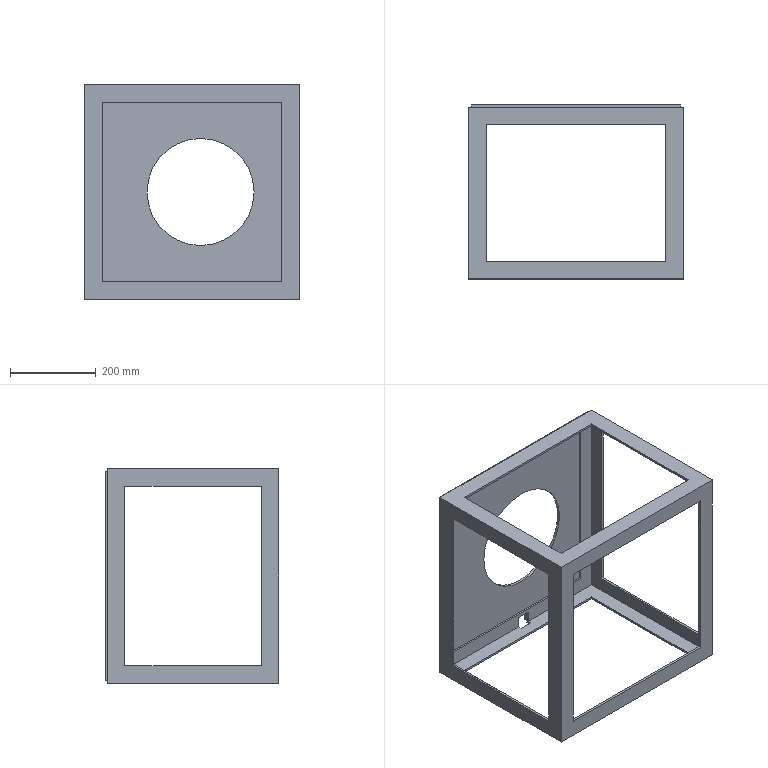Component | SolidWorks | LX-TSJ-03-1 | 1 solid | 49 faces | volume 3043684 mm3 | plane 47 | cylinder 2 | commonest cylinder face diameters 250 x2